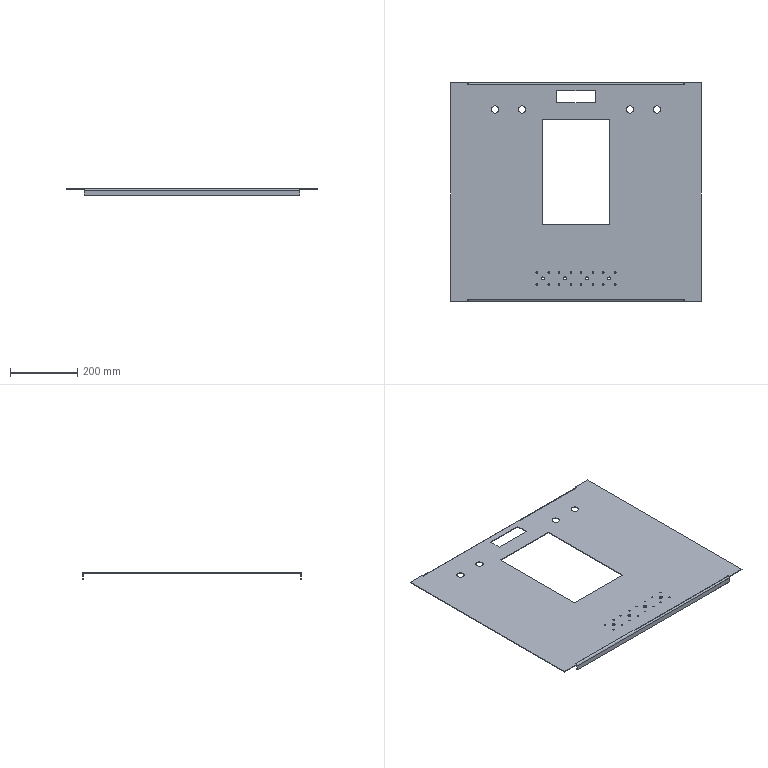Component | SolidWorks | Panel5-2 | 1 solid | 94 faces | volume 871269 mm3 | cylinder 52 | plane 42 | commonest cylinder face diameters 4.5 x32 22 x8 9 x8 11 x2 7 x2 | material Malleable Cast Iron